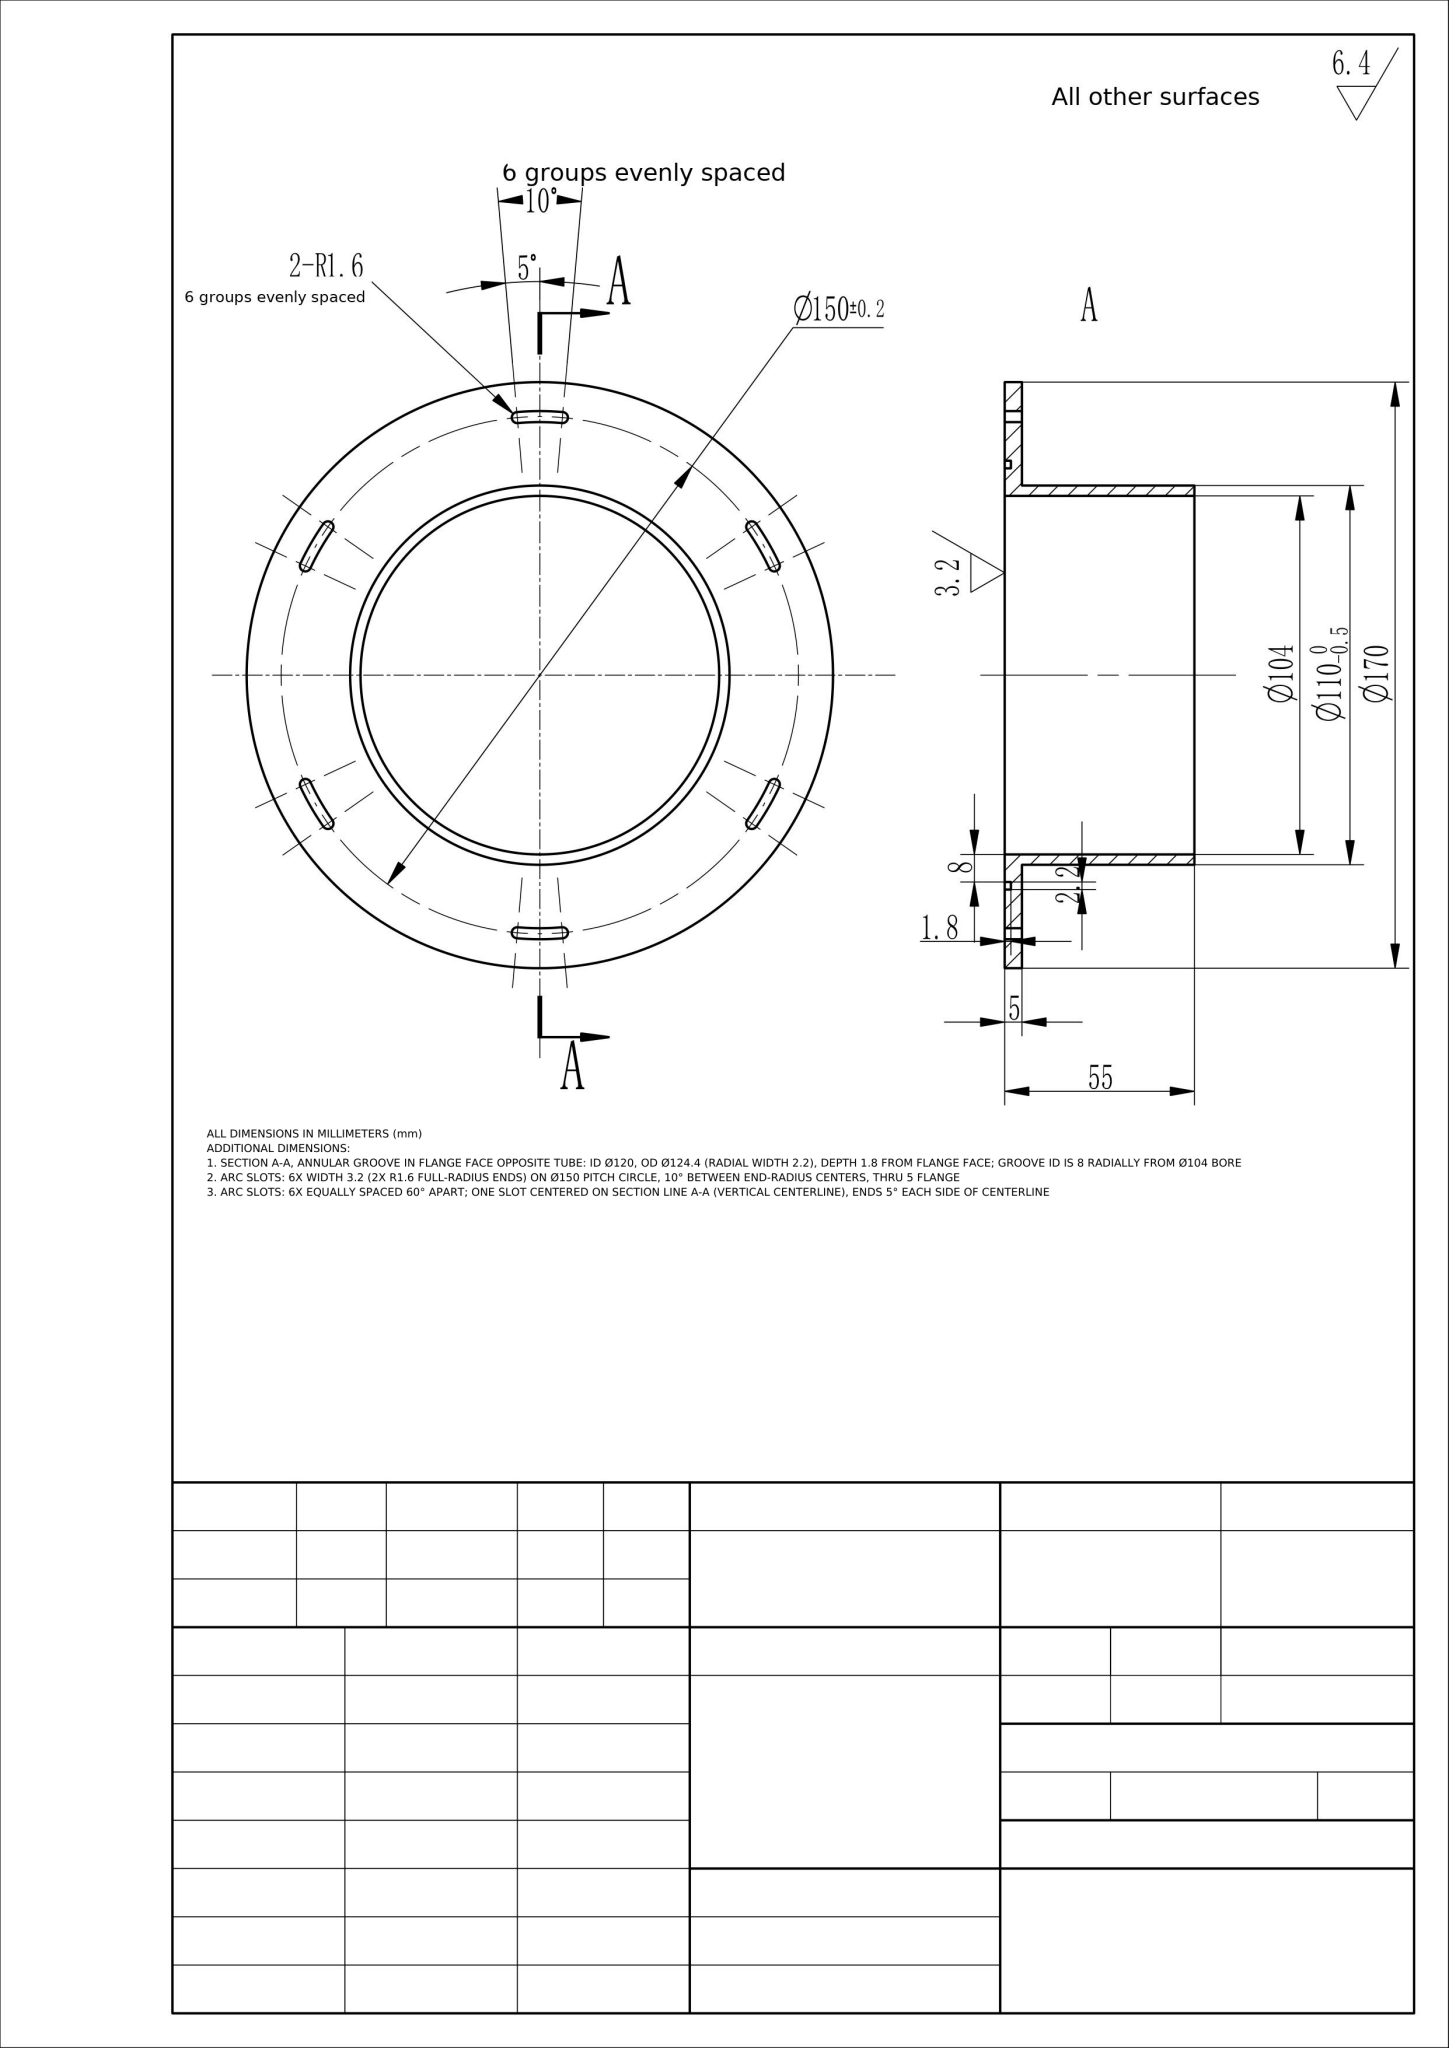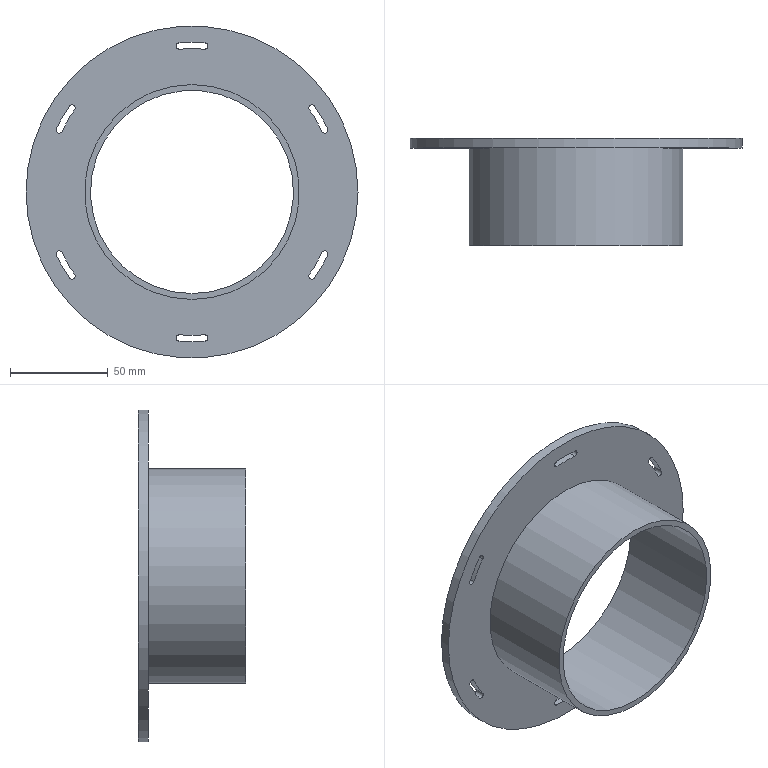Part | NX | mm | 1 solid | 34 faces | box 170 x 55 x 170 mm | volume 118420 mm3 | cylinder 29 | plane 5 | commonest cylinder face diameters 3.2 x12 146.8 x6 153.2 x6 170 x1 110 x1 104 x1 124.4 x1 120 x1